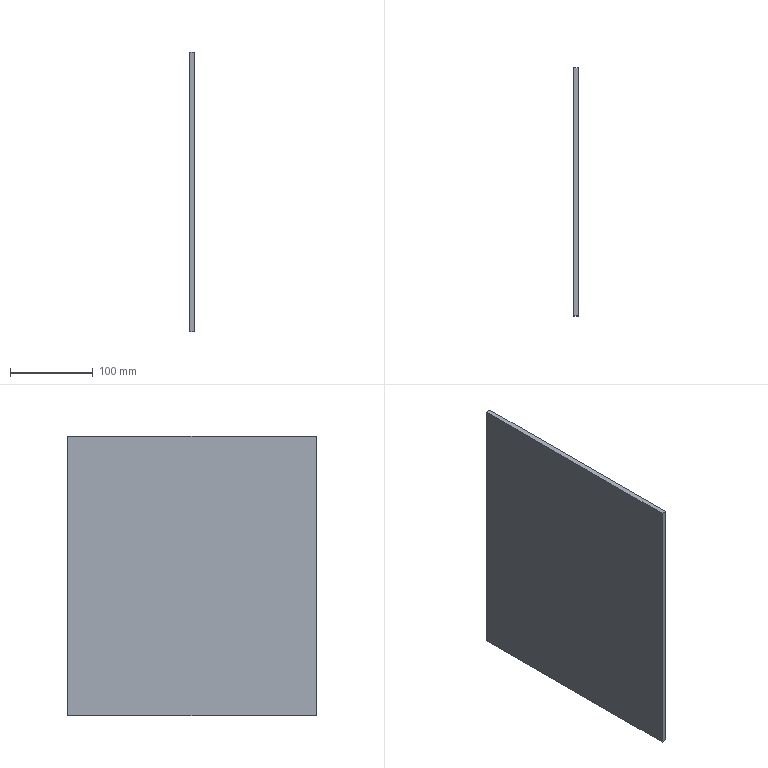Component | SolidWorks | RibPlate2-1 | 1 solid | 6 faces | box 6 x 300 x 338 mm | volume 608400 mm3 | plane 6 | material Plain Carbon Steel
STEP:
#1=COLOUR_RGB('',0.7922,0.8196,0.9333);
#2=FILL_AREA_STYLE_COLOUR('',#1);
#3=FILL_AREA_STYLE('',(#2));
#4=SURFACE_STYLE_FILL_AREA(#3);
#5=SURFACE_SIDE_STYLE('',(#4));
#6=SURFACE_STYLE_USAGE(.BOTH.,#5);
#7=PRESENTATION_STYLE_ASSIGNMENT((#6));
#8=CARTESIAN_POINT('',(69.171,126.37,79.696));
#9=VERTEX_POINT('',#8);
#10=CARTESIAN_POINT('',(69.171,126.37,66.389));
#11=VERTEX_POINT('',#10);
#12=CARTESIAN_POINT('',(69.171,126.37,66.389));
#13=DIRECTION('',(0.,-0.,-1.));
#14=VECTOR('',#13,39.37);
#15=LINE('',#12,#14);
#16=EDGE_CURVE('',#9,#11,#15,.T.);
#17=ORIENTED_EDGE('',*,*,#16,.F.);
#18=CARTESIAN_POINT('',(69.407,126.37,79.696));
#19=VERTEX_POINT('',#18);
#20=CARTESIAN_POINT('',(69.407,126.37,79.696));
#21=DIRECTION('',(-1.,-0.,0.));
#22=VECTOR('',#21,39.37);
#23=LINE('',#20,#22);
#24=EDGE_CURVE('',#19,#9,#23,.T.);
#25=ORIENTED_EDGE('',*,*,#24,.F.);
#26=CARTESIAN_POINT('',(69.407,126.37,66.389));
#27=VERTEX_POINT('',#26);
#28=CARTESIAN_POINT('',(69.407,126.37,66.389));
#29=DIRECTION('',(0.,-0.,-1.));
#30=VECTOR('',#29,39.37);
#31=LINE('',#28,#30);
#32=EDGE_CURVE('',#19,#27,#31,.T.);
#33=ORIENTED_EDGE('',*,*,#32,.T.);
#34=CARTESIAN_POINT('',(69.407,126.37,66.389));
#35=DIRECTION('',(-1.,-0.,0.));
#36=VECTOR('',#35,39.37);
#37=LINE('',#34,#36);
#38=EDGE_CURVE('',#27,#11,#37,.T.);
#39=ORIENTED_EDGE('',*,*,#38,.T.);
#40=EDGE_LOOP('',(#17,#25,#33,#39));
#41=FACE_OUTER_BOUND('',#40,.T.);
#42=CARTESIAN_POINT('',(69.407,126.37,66.389));
#43=DIRECTION('',(-0.,1.,-0.));
#44=DIRECTION('',(0.,-0.,-1.));
#45=AXIS2_PLACEMENT_3D('',#42,#43,#44);
#46=PLANE('',#45);
#47=ADVANCED_FACE('',(#41),#46,.T.);
#48=CARTESIAN_POINT('',(69.171,114.559,79.696));
#49=VERTEX_POINT('',#48);
#50=CARTESIAN_POINT('',(69.171,114.559,79.696));
#51=DIRECTION('',(-0.,1.,0.));
#52=VECTOR('',#51,39.37);
#53=LINE('',#50,#52);
#54=EDGE_CURVE('',#49,#9,#53,.T.);
#55=ORIENTED_EDGE('',*,*,#54,.F.);
#56=CARTESIAN_POINT('',(69.407,114.559,79.696));
#57=VERTEX_POINT('',#56);
#58=CARTESIAN_POINT('',(69.407,114.559,79.696));
#59=DIRECTION('',(-1.,-0.,0.));
#60=VECTOR('',#59,39.37);
#61=LINE('',#58,#60);
#62=EDGE_CURVE('',#57,#49,#61,.T.);
#63=ORIENTED_EDGE('',*,*,#62,.F.);
#64=CARTESIAN_POINT('',(69.407,114.559,79.696));
#65=DIRECTION('',(-0.,1.,0.));
#66=VECTOR('',#65,39.37);
#67=LINE('',#64,#66);
#68=EDGE_CURVE('',#57,#19,#67,.T.);
#69=ORIENTED_EDGE('',*,*,#68,.T.);
#70=ORIENTED_EDGE('',*,*,#24,.T.);
#71=EDGE_LOOP('',(#55,#63,#69,#70));
#72=FACE_OUTER_BOUND('',#71,.T.);
#73=CARTESIAN_POINT('',(69.407,114.559,79.696));
#74=DIRECTION('',(0.,0.,1.));
#75=DIRECTION('',(-0.,1.,0.));
#76=AXIS2_PLACEMENT_3D('',#73,#74,#75);
#77=PLANE('',#76);
#78=ADVANCED_FACE('',(#72),#77,.T.);
#79=CARTESIAN_POINT('',(69.171,114.559,66.389));
#80=VERTEX_POINT('',#79);
#81=CARTESIAN_POINT('',(69.171,114.559,66.389));
#82=DIRECTION('',(-0.,0.,1.));
#83=VECTOR('',#82,39.37);
#84=LINE('',#81,#83);
#85=EDGE_CURVE('',#80,#49,#84,.T.);
#86=ORIENTED_EDGE('',*,*,#85,.F.);
#87=CARTESIAN_POINT('',(69.407,114.559,66.389));
#88=VERTEX_POINT('',#87);
#89=CARTESIAN_POINT('',(69.407,114.559,66.389));
#90=DIRECTION('',(-1.,-0.,0.));
#91=VECTOR('',#90,39.37);
#92=LINE('',#89,#91);
#93=EDGE_CURVE('',#88,#80,#92,.T.);
#94=ORIENTED_EDGE('',*,*,#93,.F.);
#95=CARTESIAN_POINT('',(69.407,114.559,66.389));
#96=DIRECTION('',(-0.,0.,1.));
#97=VECTOR('',#96,39.37);
#98=LINE('',#95,#97);
#99=EDGE_CURVE('',#88,#57,#98,.T.);
#100=ORIENTED_EDGE('',*,*,#99,.T.);
#101=ORIENTED_EDGE('',*,*,#62,.T.);
#102=EDGE_LOOP('',(#86,#94,#100,#101));
#103=FACE_OUTER_BOUND('',#102,.T.);
#104=CARTESIAN_POINT('',(69.407,114.559,66.389));
#105=DIRECTION('',(0.,-1.,0.));
#106=DIRECTION('',(-0.,0.,1.));
#107=AXIS2_PLACEMENT_3D('',#104,#105,#106);
#108=PLANE('',#107);
#109=ADVANCED_FACE('',(#103),#108,.T.);
#110=CARTESIAN_POINT('',(69.171,114.559,66.389));
#111=DIRECTION('',(0.,-1.,0.));
#112=VECTOR('',#111,39.37);
#113=LINE('',#110,#112);
#114=EDGE_CURVE('',#11,#80,#113,.T.);
#115=ORIENTED_EDGE('',*,*,#114,.F.);
#116=ORIENTED_EDGE('',*,*,#38,.F.);
#117=CARTESIAN_POINT('',(69.407,114.559,66.389));
#118=DIRECTION('',(0.,-1.,0.));
#119=VECTOR('',#118,39.37);
#120=LINE('',#117,#119);
#121=EDGE_CURVE('',#27,#88,#120,.T.);
#122=ORIENTED_EDGE('',*,*,#121,.T.);
#123=ORIENTED_EDGE('',*,*,#93,.T.);
#124=EDGE_LOOP('',(#115,#116,#122,#123));
#125=FACE_OUTER_BOUND('',#124,.T.);
#126=CARTESIAN_POINT('',(69.407,114.559,66.389));
#127=DIRECTION('',(0.,0.,-1.));
#128=DIRECTION('',(0.,-1.,0.));
#129=AXIS2_PLACEMENT_3D('',#126,#127,#128);
#130=PLANE('',#129);
#131=ADVANCED_FACE('',(#125),#130,.T.);
#132=ORIENTED_EDGE('',*,*,#32,.F.);
#133=ORIENTED_EDGE('',*,*,#68,.F.);
#134=ORIENTED_EDGE('',*,*,#99,.F.);
#135=ORIENTED_EDGE('',*,*,#121,.F.);
#136=EDGE_LOOP('',(#132,#133,#134,#135));
#137=FACE_OUTER_BOUND('',#136,.T.);
#138=CARTESIAN_POINT('',(69.407,120.465,73.043));
#139=DIRECTION('',(-1.,-0.,0.));
#140=DIRECTION('',(0.,0.,1.));
#141=AXIS2_PLACEMENT_3D('',#138,#139,#140);
#142=PLANE('',#141);
#143=ADVANCED_FACE('',(#137),#142,.F.);
#144=ORIENTED_EDGE('',*,*,#16,.T.);
#145=ORIENTED_EDGE('',*,*,#114,.T.);
#146=ORIENTED_EDGE('',*,*,#85,.T.);
#147=ORIENTED_EDGE('',*,*,#54,.T.);
#148=EDGE_LOOP('',(#144,#145,#146,#147));
#149=FACE_OUTER_BOUND('',#148,.T.);
#150=CARTESIAN_POINT('',(69.171,120.465,73.043));
#151=DIRECTION('',(-1.,-0.,0.));
#152=DIRECTION('',(0.,0.,1.));
#153=AXIS2_PLACEMENT_3D('',#150,#151,#152);
#154=PLANE('',#153);
#155=ADVANCED_FACE('',(#149),#154,.T.);
#156=CLOSED_SHELL('',(#47,#78,#109,#131,#143,#155));
#157=MANIFOLD_SOLID_BREP('',#156);
#158=STYLED_ITEM('',(#7),#157);
#159=(LENGTH_UNIT()NAMED_UNIT(*)SI_UNIT($,.METRE.));
#160=LENGTH_MEASURE_WITH_UNIT(LENGTH_MEASURE(0.0254),#159);
#161=DIMENSIONAL_EXPONENTS(1.,0.,0.,0.,0.,0.,0.);
#162=(CONVERSION_BASED_UNIT('',#160)LENGTH_UNIT()NAMED_UNIT(#161));
#163=UNCERTAINTY_MEASURE_WITH_UNIT(LENGTH_MEASURE(0.00001),#162,'','');
#164=(NAMED_UNIT(*)PLANE_ANGLE_UNIT()SI_UNIT($,.RADIAN.));
#165=(NAMED_UNIT(*)SI_UNIT($,.STERADIAN.)SOLID_ANGLE_UNIT());
#166=(GEOMETRIC_REPRESENTATION_CONTEXT(3)GLOBAL_UNCERTAINTY_ASSIGNED_CONTEXT((#163))GLOBAL_UNIT_ASSIGNED_CONTEXT((#162,#164,#165))REPRESENTATION_CONTEXT('',''));
#167=MECHANICAL_DESIGN_GEOMETRIC_PRESENTATION_REPRESENTATION('',(#158),#166);
#168=PRESENTATION_LAYER_ASSIGNMENT('','',(#158));
#169=CARTESIAN_POINT('',(0.,0.,0.));
#170=DIRECTION('',(0.,0.,1.));
#171=DIRECTION('',(1.,0.,0.));
#172=AXIS2_PLACEMENT_3D('',#169,#170,#171);
#173=(LENGTH_UNIT()NAMED_UNIT(*)SI_UNIT($,.METRE.));
#174=LENGTH_MEASURE_WITH_UNIT(LENGTH_MEASURE(0.0254),#173);
#175=DIMENSIONAL_EXPONENTS(1.,0.,0.,0.,0.,0.,0.);
#176=(CONVERSION_BASED_UNIT('',#174)LENGTH_UNIT()NAMED_UNIT(#175));
#177=UNCERTAINTY_MEASURE_WITH_UNIT(LENGTH_MEASURE(0.00001),#176,'','');
#178=(NAMED_UNIT(*)PLANE_ANGLE_UNIT()SI_UNIT($,.RADIAN.));
#179=(NAMED_UNIT(*)SI_UNIT($,.STERADIAN.)SOLID_ANGLE_UNIT());
#180=(GEOMETRIC_REPRESENTATION_CONTEXT(3)GLOBAL_UNCERTAINTY_ASSIGNED_CONTEXT((#177))GLOBAL_UNIT_ASSIGNED_CONTEXT((#176,#178,#179))REPRESENTATION_CONTEXT('',''));
#181=ADVANCED_BREP_SHAPE_REPRESENTATION('',(#157,#172),#180);